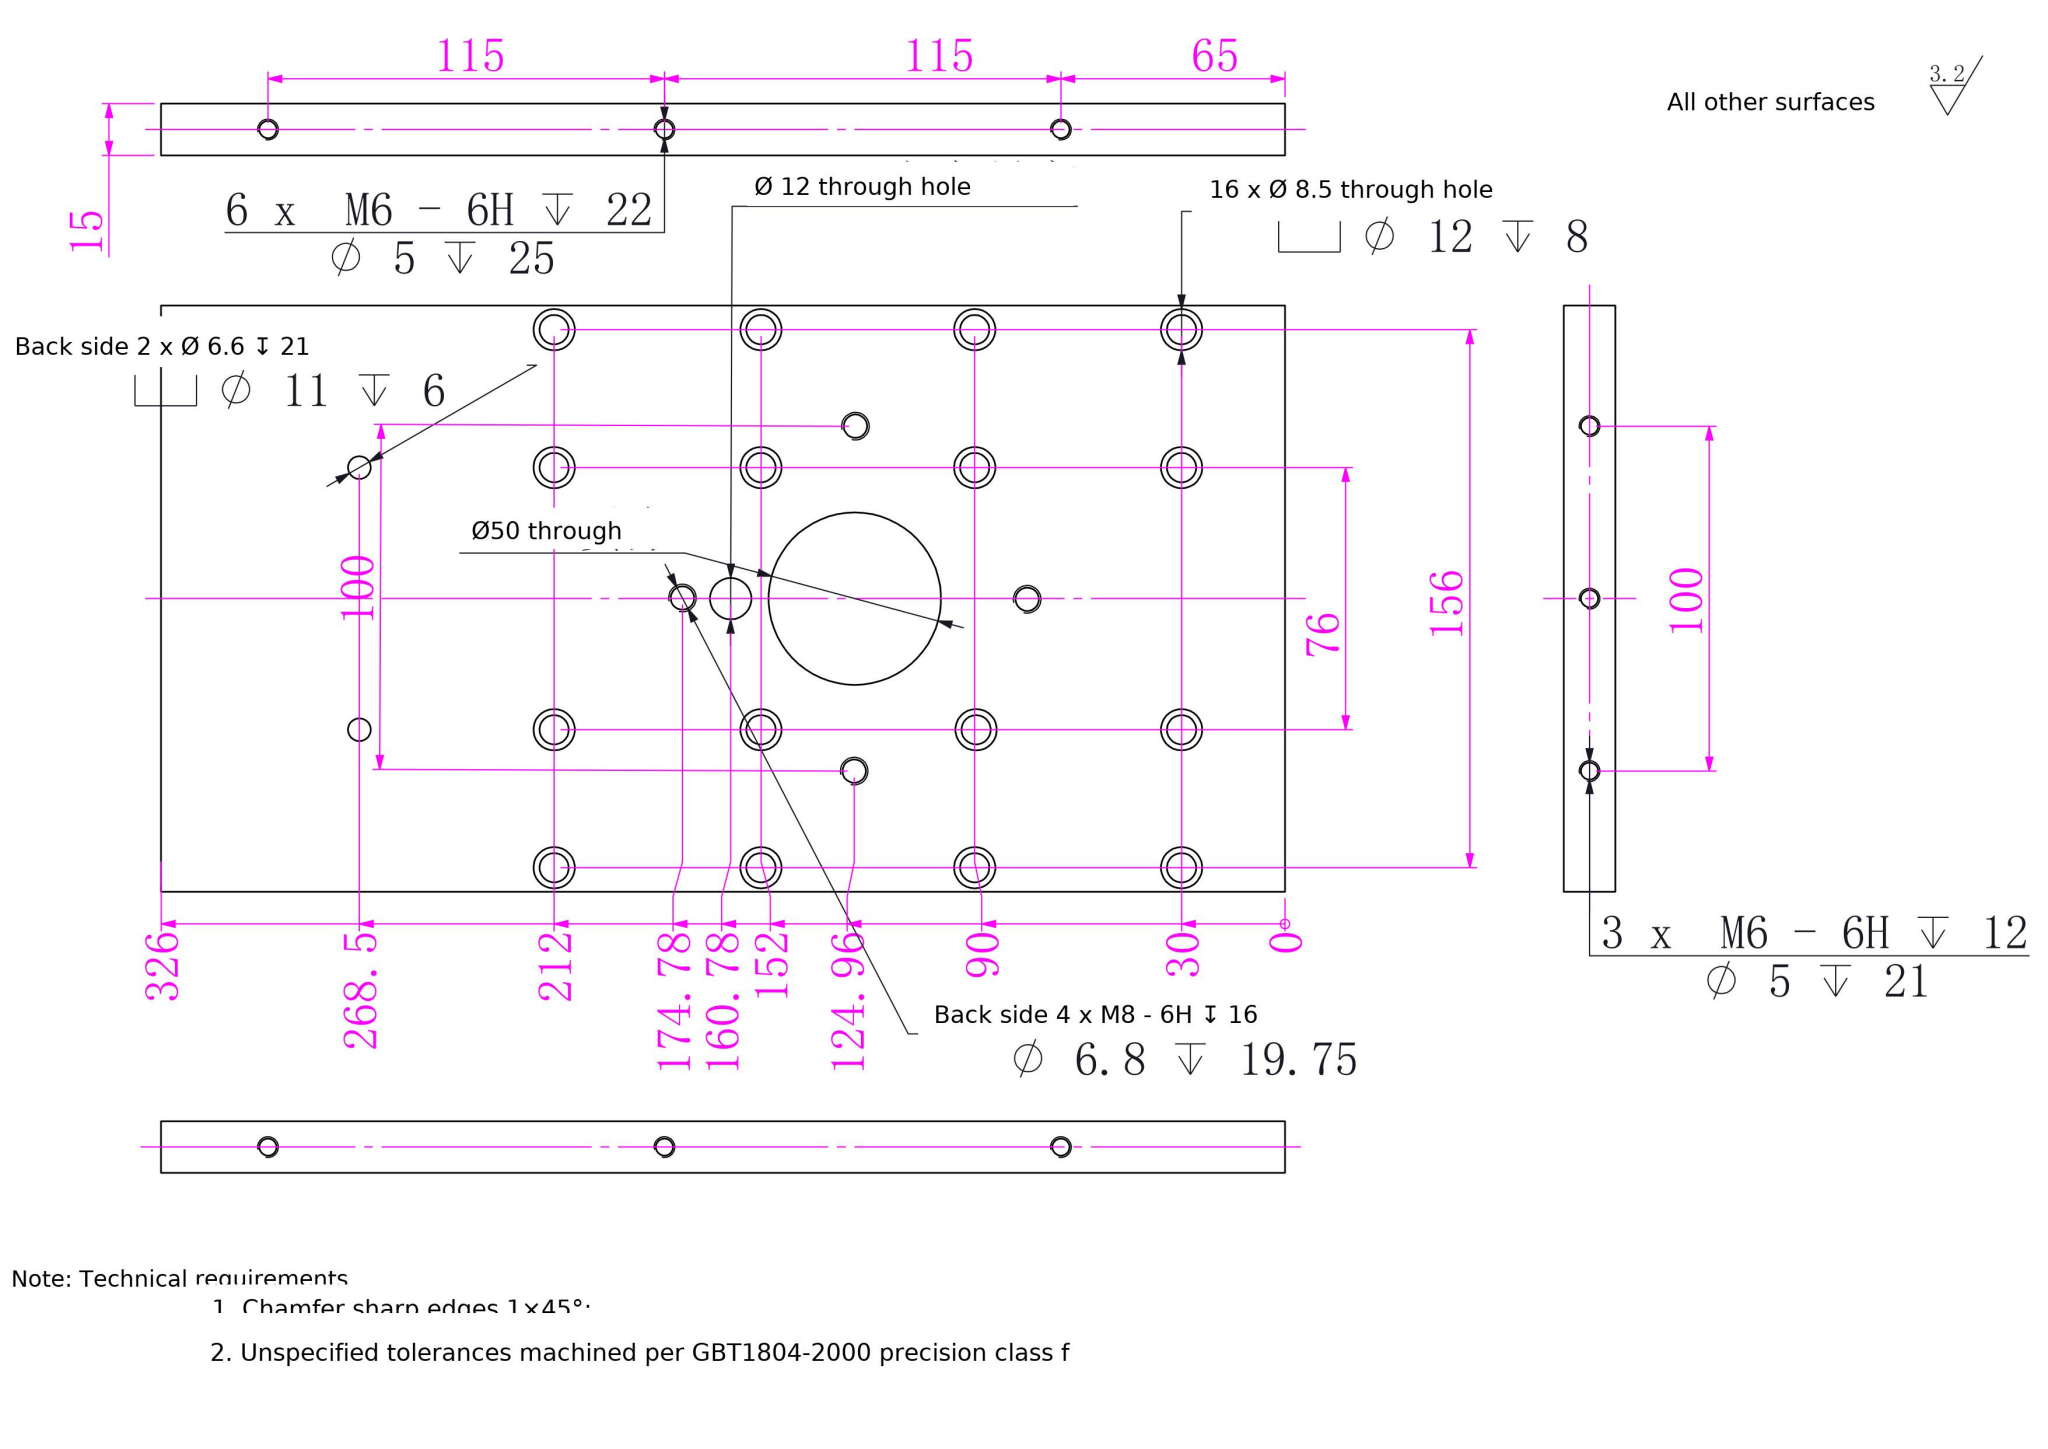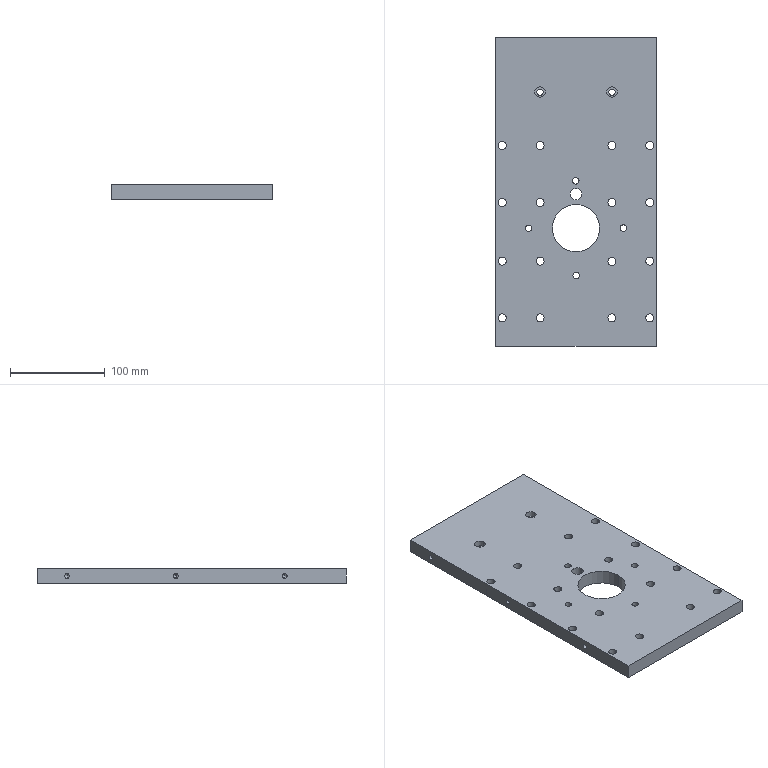Part | SolidWorks | mm | 1 solid | 144 faces | box 170 x 326 x 15 mm | volume 771113 mm3 | cylinder 102 | plane 24 | cone 18 | commonest cylinder face diameters 12 x34 8.5 x32 5 x18 6.8 x8 11 x4 6.6 x4 50 x2